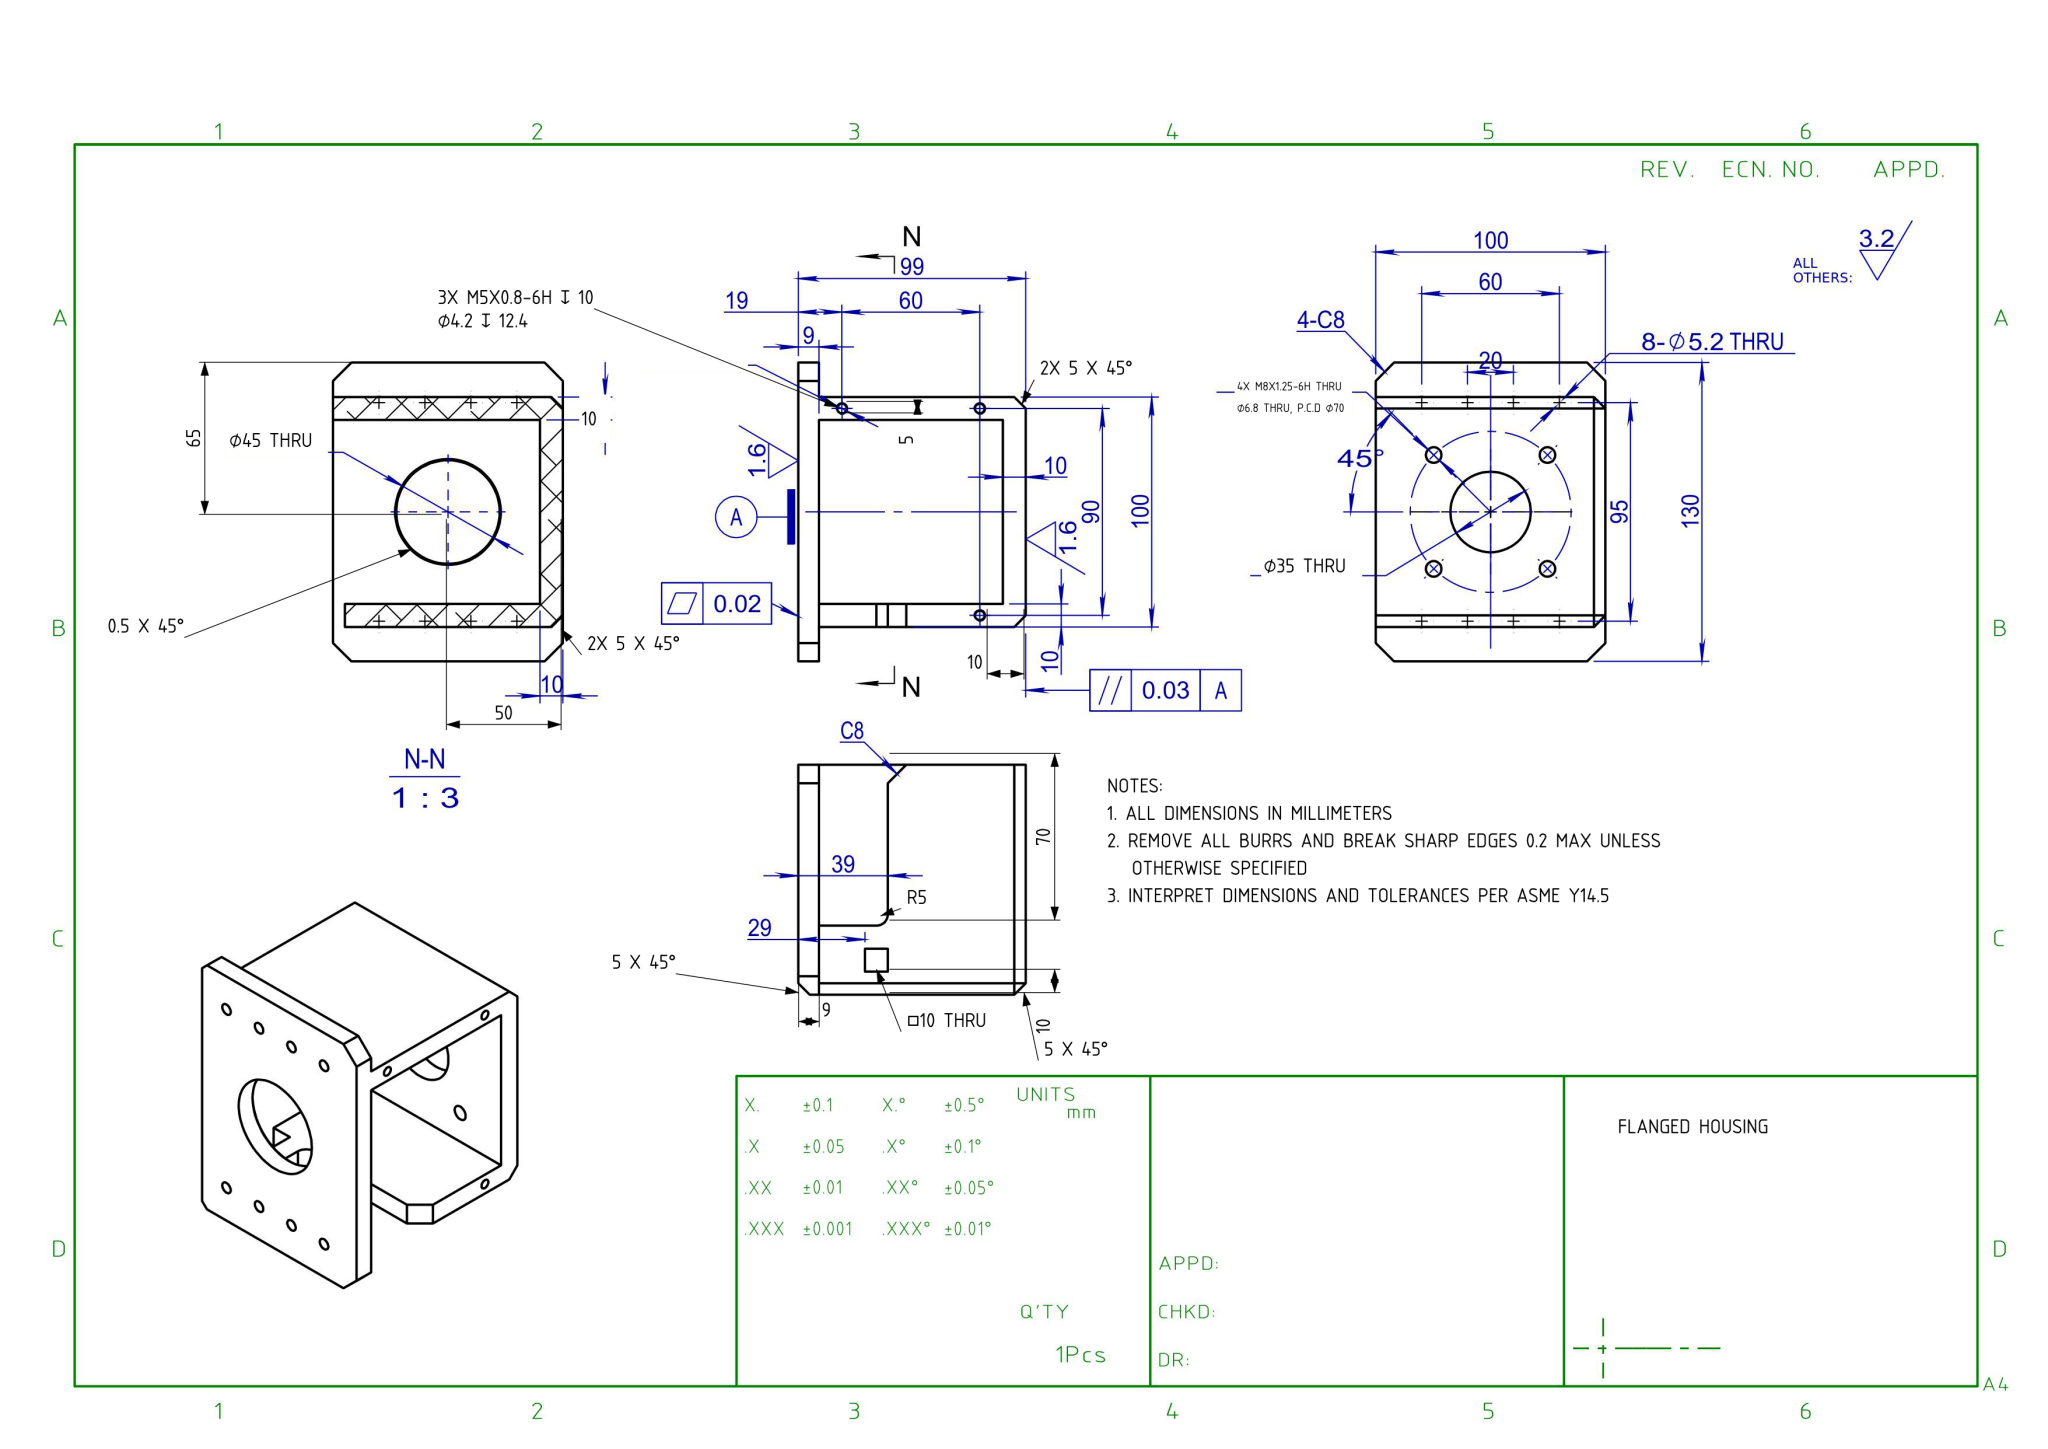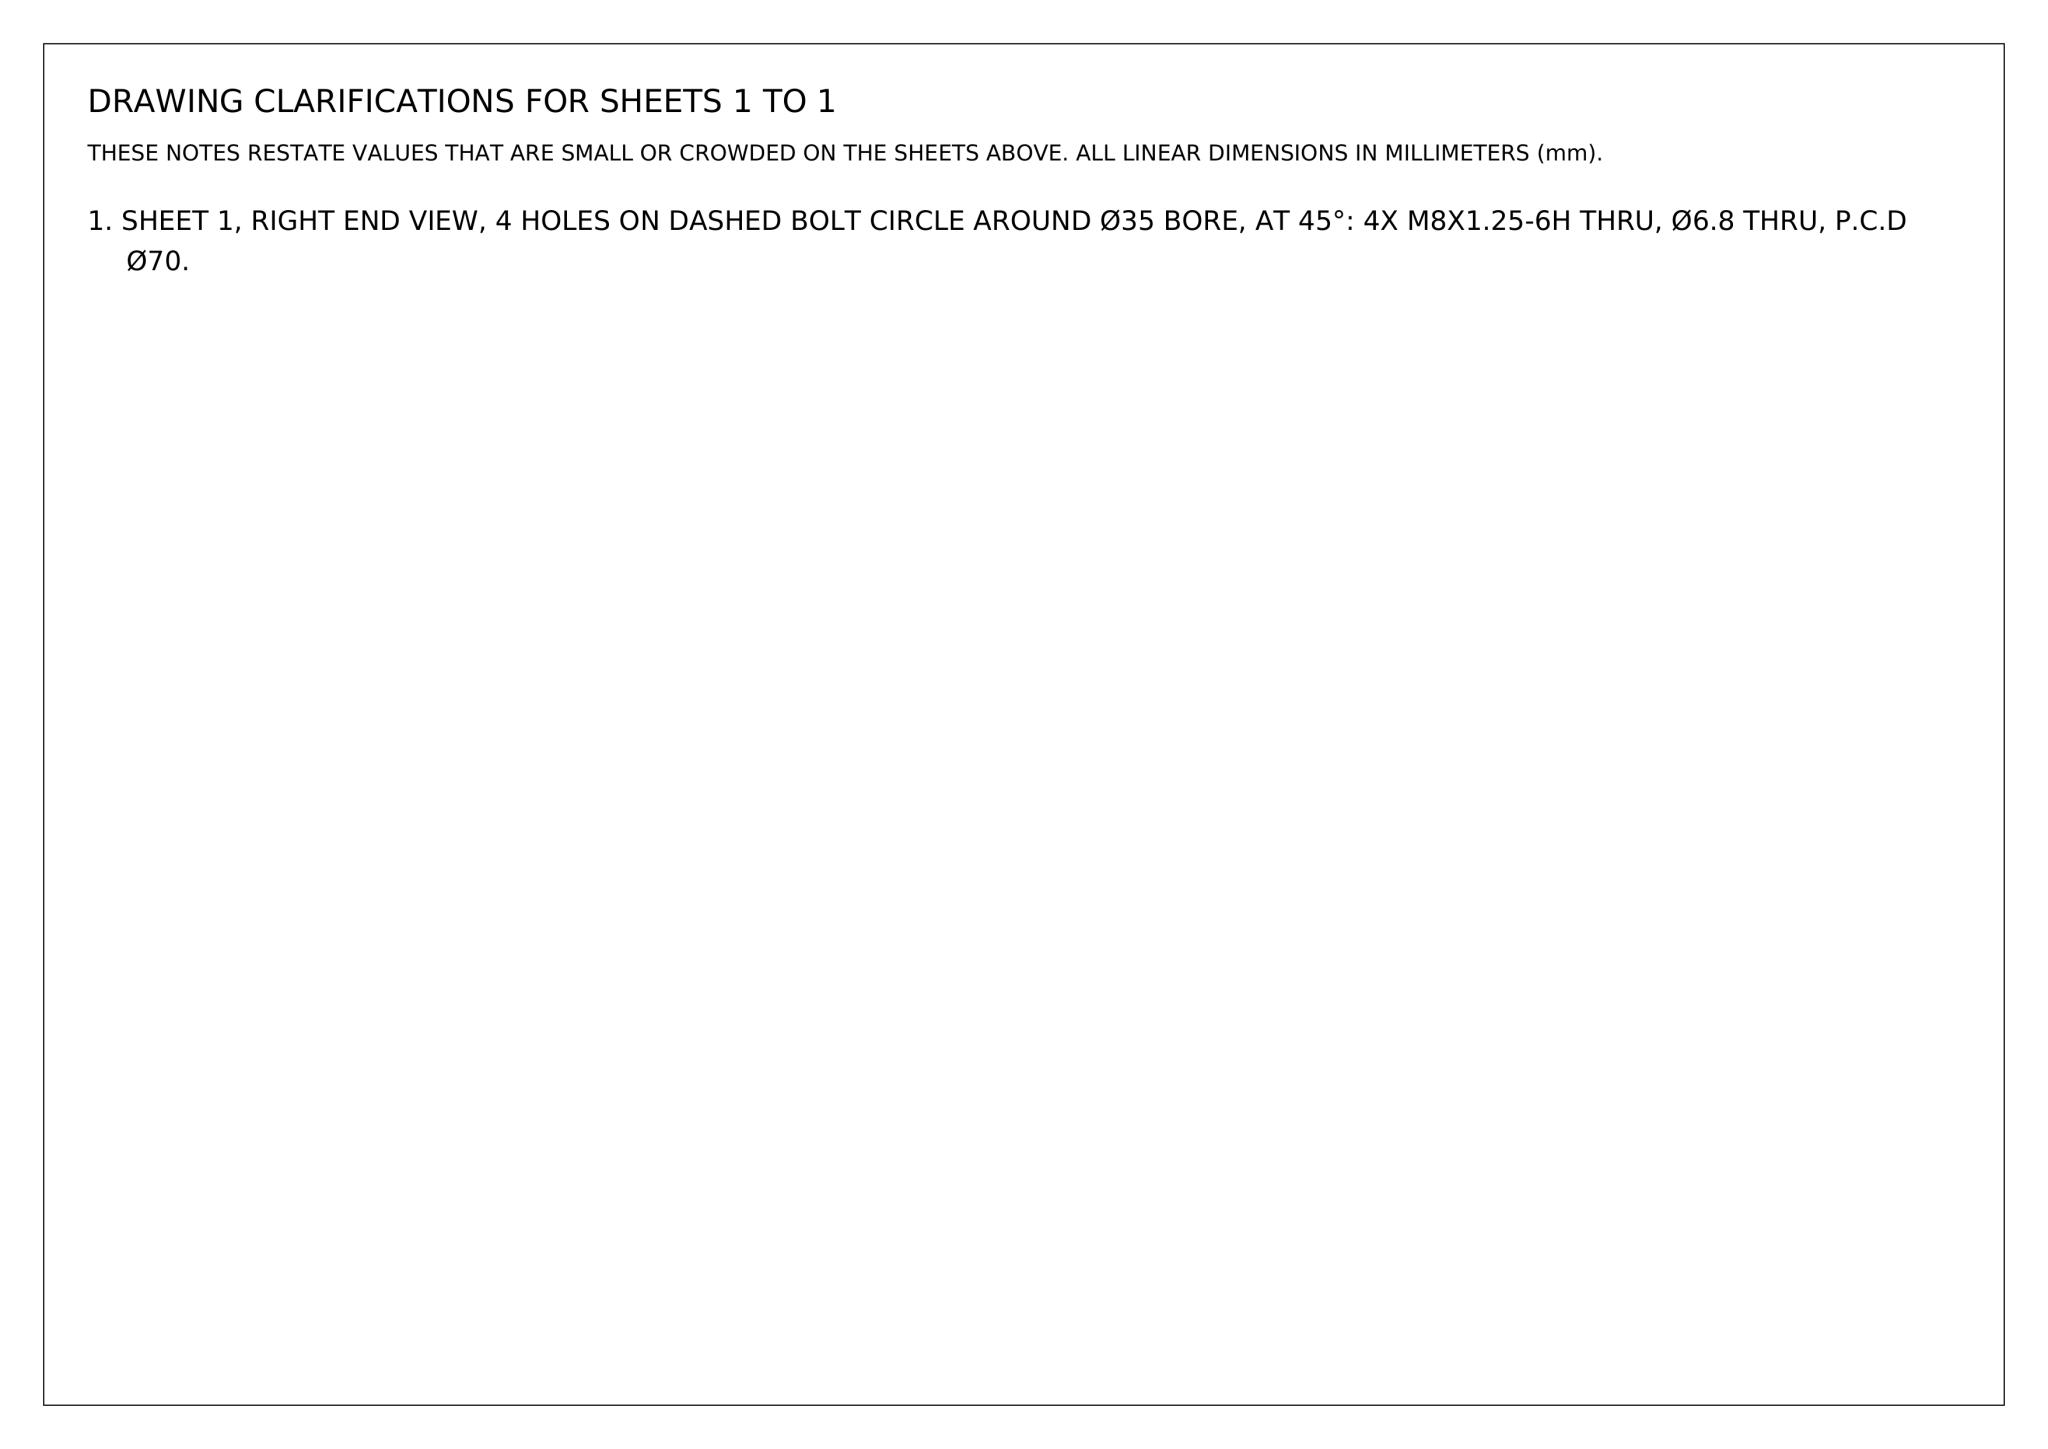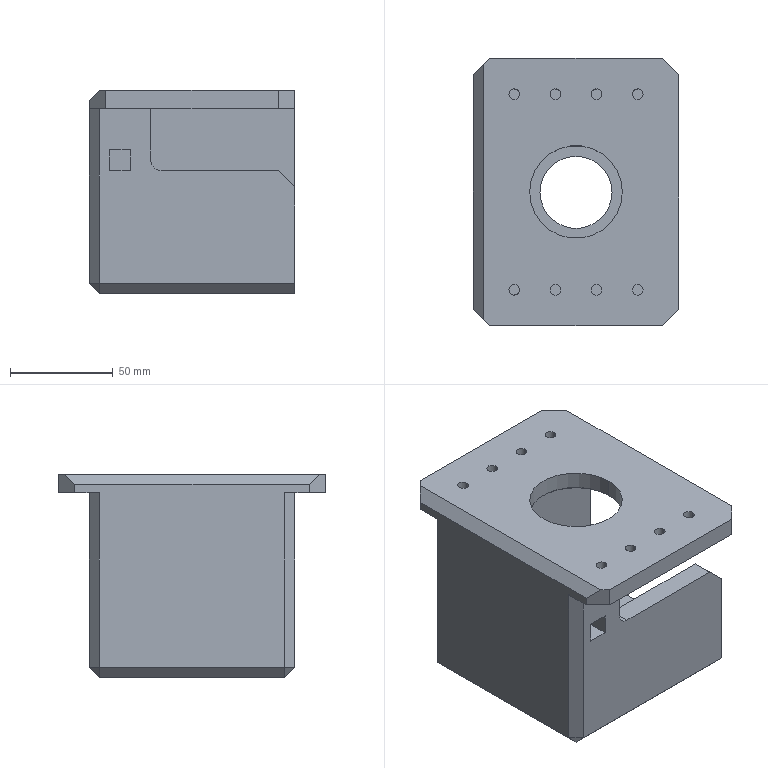Part | NX | mm | 1 solid | 80 faces | box 100 x 130 x 99 mm | volume 382814 mm3 | plane 37 | cylinder 35 | cone 8 | commonest cylinder face diameters 5.2 x16 6.8 x8 4.2 x6 35 x2 45 x2 10 x1